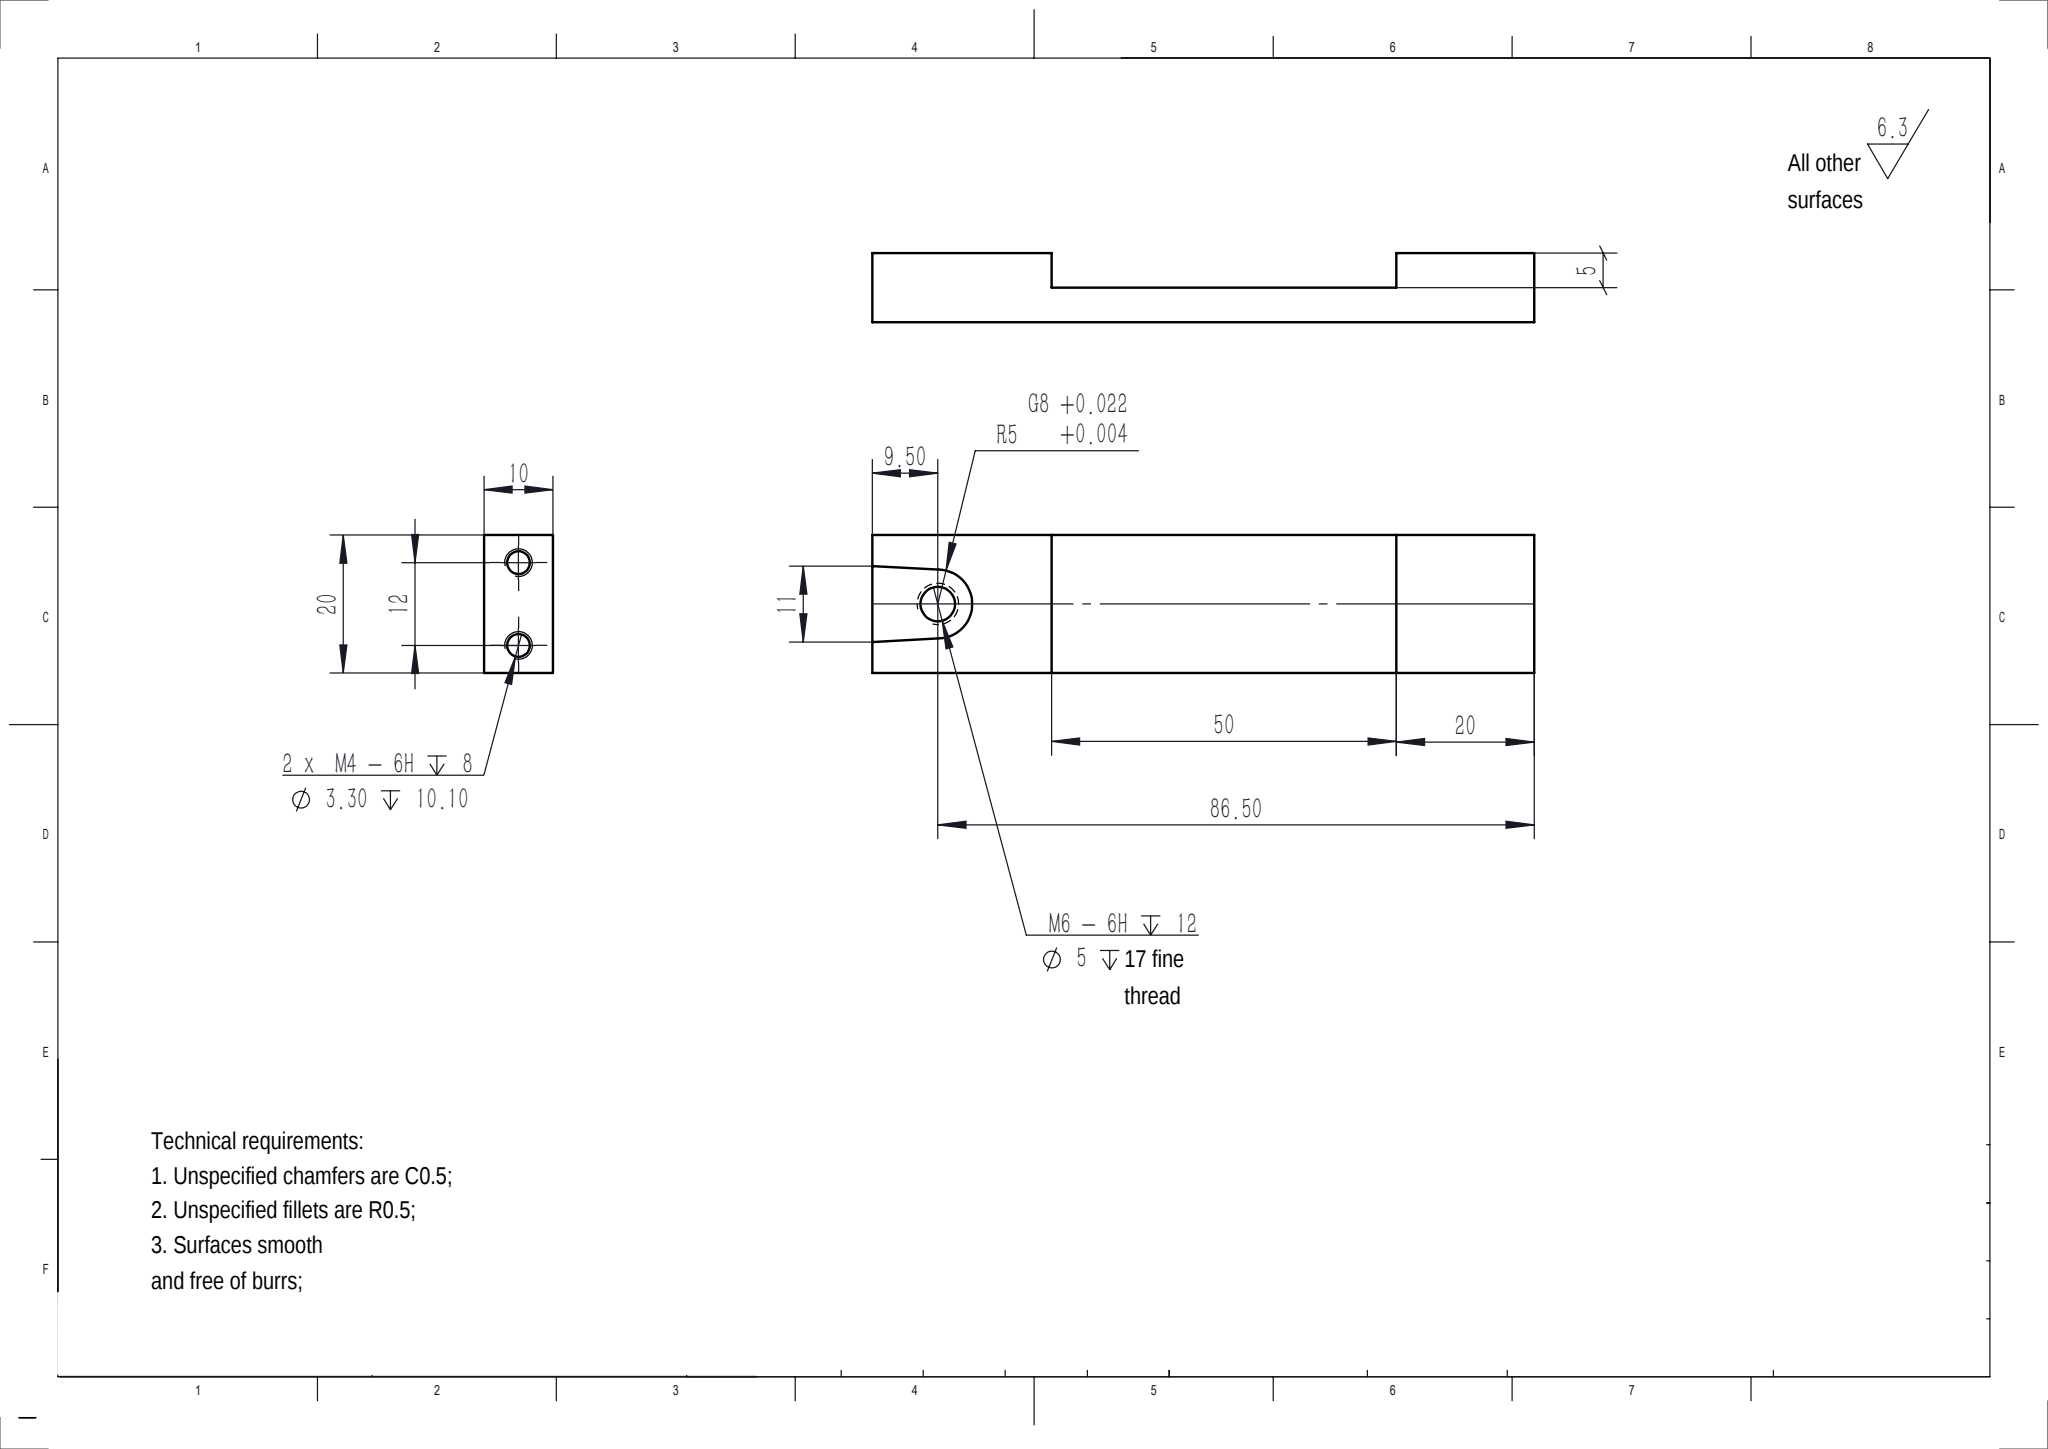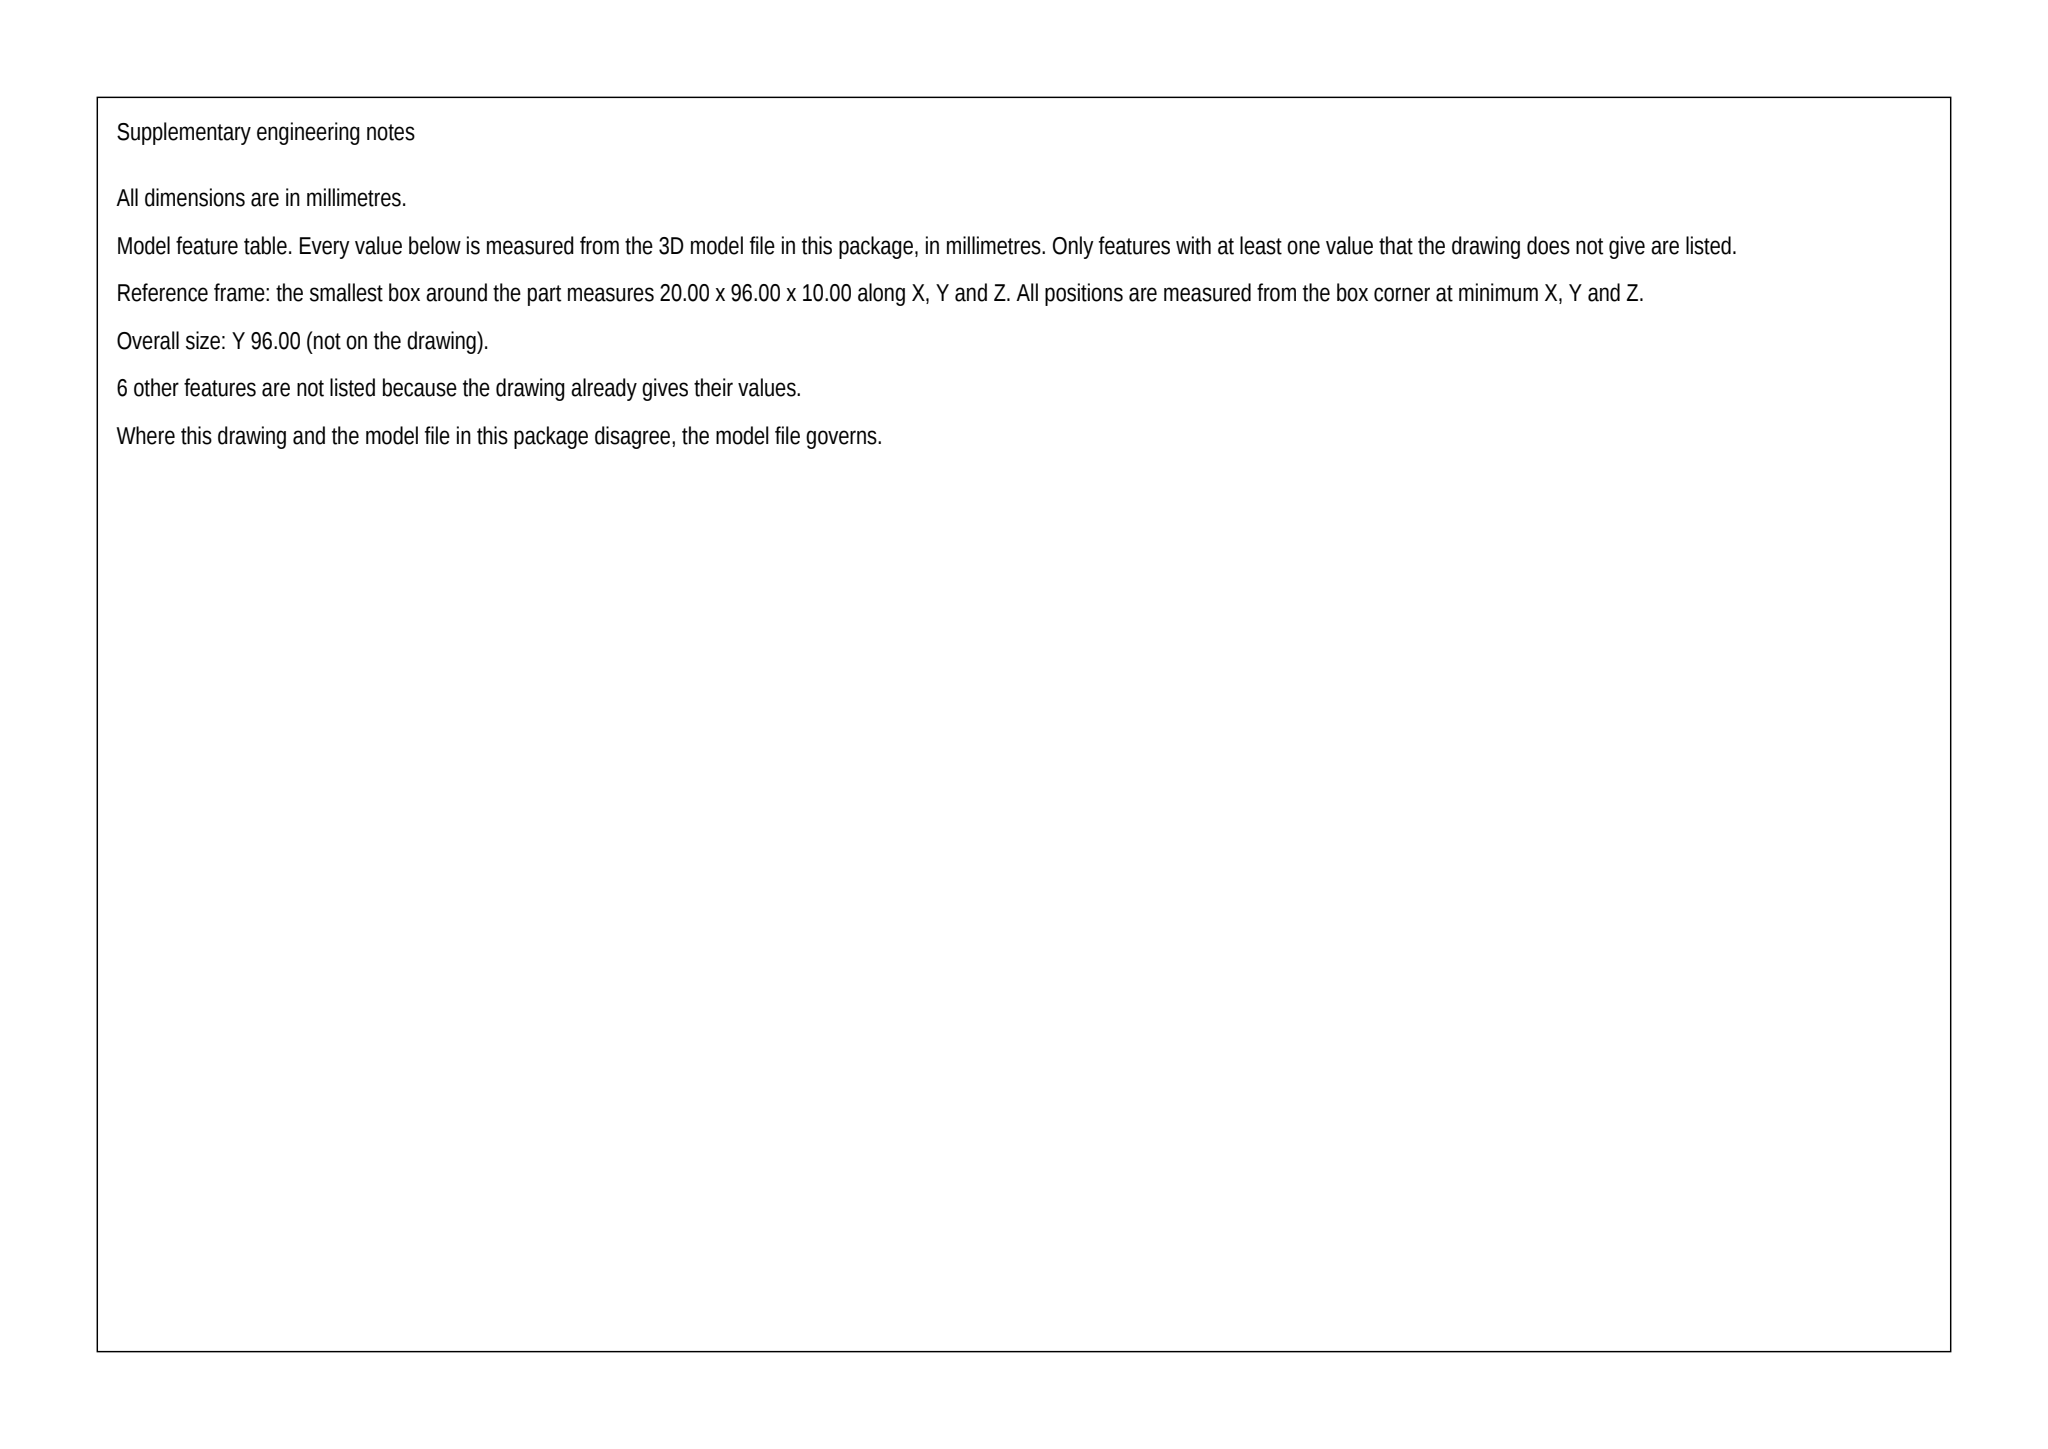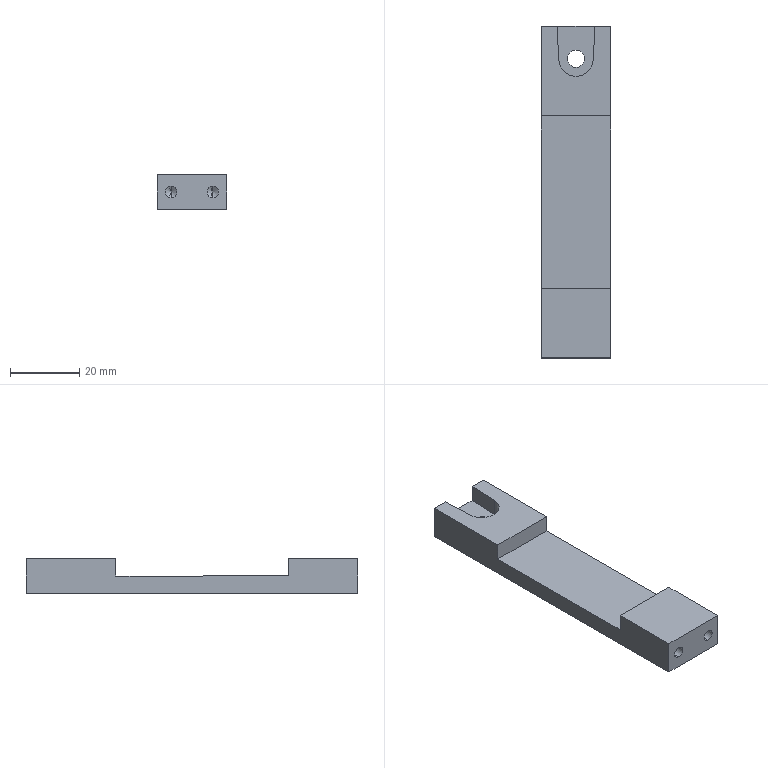Part | SolidWorks | mm | 1 solid | 24 faces | box 20 x 96 x 10 mm | volume 13228 mm3 | plane 13 | cylinder 7 | cone 4 | commonest cylinder face diameters 3.3 x4 5 x2 10 x1
build123d program:
from build123d import *

# Parameters (mm, degrees)
SKETCH1_W             = 20
SKETCH1_H             = 96
BOSS_EXTRUDE1_DEPTH   = 10
CUT_EXTRUDE1_DEPTH    = 5
M4_TAPPED_HOLE1_D     = 3.3
M4_TAPPED_HOLE1_DEPTH = 10.1
M4_TAPPED_HOLE1_TIP   = 0.9914
CUT_EXTRUDE3_DEPTH    = 5
M6_TAPPED_HOLE1_D     = 5
M6_TAPPED_HOLE1_DEPTH = 17
M6_TAPPED_HOLE1_TIP   = 1.502
SKETCH10_W            = 5
SKETCH10_H            = 50
CUT_EXTRUDE4_DEPTH    = 53.953


with BuildPart() as part:
    # Sketch1 → Boss-Extrude1 (new body)
    with BuildSketch(Plane.XY):
        Rectangle(SKETCH1_W, SKETCH1_H)
    extrude(amount=BOSS_EXTRUDE1_DEPTH)

    # Sketch2 → Cut-Extrude1 (cut)
    with BuildSketch(Plane.XY.offset(10)):
        with BuildLine():
            Line((-5, 48), (5, 48))
            Line((5, 48), (5, 38.5))
            ThreePointArc((5, 38.5), (0, 33.5), (-5, 38.5))
            Line((-5, 38.5), (-5, 48))
        make_face()
    extrude(amount=-CUT_EXTRUDE1_DEPTH, mode=Mode.SUBTRACT)

    # M4 Tapped Hole1
    with Locations(Plane(origin=(0, -48, 0), x_dir=(-1, 0, 0), z_dir=(0, -1, 0))):
        with Locations((6, -5), (-6, -5)):
            Hole(M4_TAPPED_HOLE1_D / 2, depth=M4_TAPPED_HOLE1_DEPTH)
            with Locations((0, 0, -(M4_TAPPED_HOLE1_DEPTH + M4_TAPPED_HOLE1_TIP / 2))):  # 118° drill point
                Cone(0, M4_TAPPED_HOLE1_D / 2, M4_TAPPED_HOLE1_TIP, mode=Mode.SUBTRACT)

    # Sketch7 → Cut-Extrude3 (cut)
    with BuildSketch(Plane.XY.offset(10)):
        Polygon((-5, 38.5), (-5.5, 48), (5.5, 48), (5, 38.5), align=None)
    extrude(amount=-CUT_EXTRUDE3_DEPTH, mode=Mode.SUBTRACT)

    # M6 Tapped Hole1
    with Locations(Plane(origin=(0, 0, 0), x_dir=(-1, 0, 0), z_dir=(0, 0, -1))):
        with Locations((0, 38.5)):
            Hole(M6_TAPPED_HOLE1_D / 2, depth=M6_TAPPED_HOLE1_DEPTH)
            with Locations((0, 0, -(M6_TAPPED_HOLE1_DEPTH + M6_TAPPED_HOLE1_TIP / 2))):  # 118° drill point
                Cone(0, M6_TAPPED_HOLE1_D / 2, M6_TAPPED_HOLE1_TIP, mode=Mode.SUBTRACT)

    # Sketch10 → Cut-Extrude4 (cut, through all)
    with BuildSketch(Plane.ZY.offset(10)):
        with Locations((7.5, -3)):
            Rectangle(SKETCH10_W, SKETCH10_H)
    extrude(amount=-CUT_EXTRUDE4_DEPTH, mode=Mode.SUBTRACT)


solid = part.part
STEP:
#1=CARTESIAN_POINT('',(-2.5,38.5,5.));
#2=VERTEX_POINT('',#1);
#3=CARTESIAN_POINT('',(2.5,38.5,5.));
#4=VERTEX_POINT('',#3);
#5=CARTESIAN_POINT('',(0.,38.5,5.));
#6=DIRECTION('',(0.,0.,1.));
#7=DIRECTION('',(1.,0.,0.));
#8=AXIS2_PLACEMENT_3D('',#5,#6,#7);
#9=CIRCLE('',#8,2.5);
#10=EDGE_CURVE('',#2,#4,#9,.T.);
#11=ORIENTED_EDGE('',*,*,#10,.T.);
#12=CARTESIAN_POINT('',(2.5,38.5,0.));
#13=VERTEX_POINT('',#12);
#14=CARTESIAN_POINT('',(2.5,38.5,0.));
#15=DIRECTION('',(0.,0.,-1.));
#16=VECTOR('',#15,1000.);
#17=LINE('',#14,#16);
#18=EDGE_CURVE('',#4,#13,#17,.T.);
#19=ORIENTED_EDGE('',*,*,#18,.T.);
#20=CARTESIAN_POINT('',(-2.5,38.5,0.));
#21=VERTEX_POINT('',#20);
#22=CARTESIAN_POINT('',(0.,38.5,0.));
#23=DIRECTION('',(0.,0.,-1.));
#24=DIRECTION('',(-1.,0.,0.));
#25=AXIS2_PLACEMENT_3D('',#22,#23,#24);
#26=CIRCLE('',#25,2.5);
#27=EDGE_CURVE('',#13,#21,#26,.T.);
#28=ORIENTED_EDGE('',*,*,#27,.T.);
#29=CARTESIAN_POINT('',(-2.5,38.5,0.));
#30=DIRECTION('',(0.,0.,-1.));
#31=VECTOR('',#30,1000.);
#32=LINE('',#29,#31);
#33=EDGE_CURVE('',#2,#21,#32,.T.);
#34=ORIENTED_EDGE('',*,*,#33,.F.);
#35=EDGE_LOOP('',(#11,#19,#28,#34));
#36=FACE_OUTER_BOUND('',#35,.T.);
#37=CARTESIAN_POINT('',(0.,38.5,0.));
#38=DIRECTION('',(0.,0.,-1.));
#39=DIRECTION('',(-1.,0.,0.));
#40=AXIS2_PLACEMENT_3D('',#37,#38,#39);
#41=CYLINDRICAL_SURFACE('',#40,2.5);
#42=ADVANCED_FACE('',(#36),#41,.F.);
#43=CARTESIAN_POINT('',(-6.,-37.9,6.65));
#44=VERTEX_POINT('',#43);
#45=CARTESIAN_POINT('',(-6.,-37.9,3.35));
#46=VERTEX_POINT('',#45);
#47=CARTESIAN_POINT('',(-6.,-37.9,5.));
#48=DIRECTION('',(0.,-1.,0.));
#49=DIRECTION('',(0.,0.,-1.));
#50=AXIS2_PLACEMENT_3D('',#47,#48,#49);
#51=CIRCLE('',#50,1.65);
#52=EDGE_CURVE('',#44,#46,#51,.T.);
#53=ORIENTED_EDGE('',*,*,#52,.F.);
#54=CARTESIAN_POINT('',(-6.,-48.,6.65));
#55=VERTEX_POINT('',#54);
#56=CARTESIAN_POINT('',(-6.,-48.,6.65));
#57=DIRECTION('',(0.,-1.,0.));
#58=VECTOR('',#57,1000.);
#59=LINE('',#56,#58);
#60=EDGE_CURVE('',#44,#55,#59,.T.);
#61=ORIENTED_EDGE('',*,*,#60,.T.);
#62=CARTESIAN_POINT('',(-6.,-48.,3.35));
#63=VERTEX_POINT('',#62);
#64=CARTESIAN_POINT('',(-6.,-48.,5.));
#65=DIRECTION('',(0.,-1.,0.));
#66=DIRECTION('',(0.,0.,-1.));
#67=AXIS2_PLACEMENT_3D('',#64,#65,#66);
#68=CIRCLE('',#67,1.65);
#69=EDGE_CURVE('',#55,#63,#68,.T.);
#70=ORIENTED_EDGE('',*,*,#69,.T.);
#71=CARTESIAN_POINT('',(-6.,-48.,3.35));
#72=DIRECTION('',(0.,-1.,0.));
#73=VECTOR('',#72,1000.);
#74=LINE('',#71,#73);
#75=EDGE_CURVE('',#46,#63,#74,.T.);
#76=ORIENTED_EDGE('',*,*,#75,.F.);
#77=EDGE_LOOP('',(#53,#61,#70,#76));
#78=FACE_OUTER_BOUND('',#77,.T.);
#79=CARTESIAN_POINT('',(-6.,-48.,5.));
#80=DIRECTION('',(0.,-1.,0.));
#81=DIRECTION('',(0.,0.,-1.));
#82=AXIS2_PLACEMENT_3D('',#79,#80,#81);
#83=CYLINDRICAL_SURFACE('',#82,1.65);
#84=ADVANCED_FACE('',(#78),#83,.F.);
#85=CARTESIAN_POINT('',(-6.,-36.909,5.));
#86=VERTEX_POINT('',#85);
#87=CARTESIAN_POINT('',(-6.,-37.9,3.35));
#88=DIRECTION('',(0.,-0.515,-0.8572));
#89=VECTOR('',#88,1000.);
#90=LINE('',#87,#89);
#91=EDGE_CURVE('',#86,#46,#90,.T.);
#92=ORIENTED_EDGE('',*,*,#91,.F.);
#93=CARTESIAN_POINT('',(-6.,-37.9,6.65));
#94=DIRECTION('',(0.,-0.515,0.8572));
#95=VECTOR('',#94,1000.);
#96=LINE('',#93,#95);
#97=EDGE_CURVE('',#86,#44,#96,.T.);
#98=ORIENTED_EDGE('',*,*,#97,.T.);
#99=ORIENTED_EDGE('',*,*,#52,.T.);
#100=EDGE_LOOP('',(#92,#98,#99));
#101=FACE_OUTER_BOUND('',#100,.T.);
#102=CARTESIAN_POINT('',(-6.,-37.9,5.));
#103=DIRECTION('',(0.,-1.,0.));
#104=DIRECTION('',(0.,0.,-1.));
#105=AXIS2_PLACEMENT_3D('',#102,#103,#104);
#106=CONICAL_SURFACE('',#105,1.65,1.03);
#107=ADVANCED_FACE('',(#101),#106,.F.);
#108=CARTESIAN_POINT('',(6.,-37.9,6.65));
#109=VERTEX_POINT('',#108);
#110=CARTESIAN_POINT('',(6.,-37.9,3.35));
#111=VERTEX_POINT('',#110);
#112=CARTESIAN_POINT('',(6.,-37.9,5.));
#113=DIRECTION('',(0.,-1.,0.));
#114=DIRECTION('',(0.,0.,-1.));
#115=AXIS2_PLACEMENT_3D('',#112,#113,#114);
#116=CIRCLE('',#115,1.65);
#117=EDGE_CURVE('',#109,#111,#116,.T.);
#118=ORIENTED_EDGE('',*,*,#117,.F.);
#119=CARTESIAN_POINT('',(6.,-48.,6.65));
#120=VERTEX_POINT('',#119);
#121=CARTESIAN_POINT('',(6.,-48.,6.65));
#122=DIRECTION('',(0.,-1.,0.));
#123=VECTOR('',#122,1000.);
#124=LINE('',#121,#123);
#125=EDGE_CURVE('',#109,#120,#124,.T.);
#126=ORIENTED_EDGE('',*,*,#125,.T.);
#127=CARTESIAN_POINT('',(6.,-48.,3.35));
#128=VERTEX_POINT('',#127);
#129=CARTESIAN_POINT('',(6.,-48.,5.));
#130=DIRECTION('',(0.,-1.,0.));
#131=DIRECTION('',(0.,0.,-1.));
#132=AXIS2_PLACEMENT_3D('',#129,#130,#131);
#133=CIRCLE('',#132,1.65);
#134=EDGE_CURVE('',#120,#128,#133,.T.);
#135=ORIENTED_EDGE('',*,*,#134,.T.);
#136=CARTESIAN_POINT('',(6.,-48.,3.35));
#137=DIRECTION('',(0.,-1.,0.));
#138=VECTOR('',#137,1000.);
#139=LINE('',#136,#138);
#140=EDGE_CURVE('',#111,#128,#139,.T.);
#141=ORIENTED_EDGE('',*,*,#140,.F.);
#142=EDGE_LOOP('',(#118,#126,#135,#141));
#143=FACE_OUTER_BOUND('',#142,.T.);
#144=CARTESIAN_POINT('',(6.,-48.,5.));
#145=DIRECTION('',(0.,-1.,0.));
#146=DIRECTION('',(0.,0.,-1.));
#147=AXIS2_PLACEMENT_3D('',#144,#145,#146);
#148=CYLINDRICAL_SURFACE('',#147,1.65);
#149=ADVANCED_FACE('',(#143),#148,.F.);
#150=CARTESIAN_POINT('',(6.,-36.909,5.));
#151=VERTEX_POINT('',#150);
#152=CARTESIAN_POINT('',(6.,-37.9,3.35));
#153=DIRECTION('',(0.,-0.515,-0.8572));
#154=VECTOR('',#153,1000.);
#155=LINE('',#152,#154);
#156=EDGE_CURVE('',#151,#111,#155,.T.);
#157=ORIENTED_EDGE('',*,*,#156,.F.);
#158=CARTESIAN_POINT('',(6.,-37.9,6.65));
#159=DIRECTION('',(0.,-0.515,0.8572));
#160=VECTOR('',#159,1000.);
#161=LINE('',#158,#160);
#162=EDGE_CURVE('',#151,#109,#161,.T.);
#163=ORIENTED_EDGE('',*,*,#162,.T.);
#164=ORIENTED_EDGE('',*,*,#117,.T.);
#165=EDGE_LOOP('',(#157,#163,#164));
#166=FACE_OUTER_BOUND('',#165,.T.);
#167=CARTESIAN_POINT('',(6.,-37.9,5.));
#168=DIRECTION('',(0.,-1.,0.));
#169=DIRECTION('',(0.,0.,-1.));
#170=AXIS2_PLACEMENT_3D('',#167,#168,#169);
#171=CONICAL_SURFACE('',#170,1.65,1.03);
#172=ADVANCED_FACE('',(#166),#171,.F.);
#173=CARTESIAN_POINT('',(10.,-28.,10.));
#174=VERTEX_POINT('',#173);
#175=CARTESIAN_POINT('',(-10.,-28.,10.));
#176=VERTEX_POINT('',#175);
#177=CARTESIAN_POINT('',(10.,-28.,10.));
#178=DIRECTION('',(-1.,-0.,0.));
#179=VECTOR('',#178,1000.);
#180=LINE('',#177,#179);
#181=EDGE_CURVE('',#174,#176,#180,.T.);
#182=ORIENTED_EDGE('',*,*,#181,.T.);
#183=CARTESIAN_POINT('',(-10.,-48.,10.));
#184=VERTEX_POINT('',#183);
#185=CARTESIAN_POINT('',(-10.,48.,10.));
#186=DIRECTION('',(0.,-1.,0.));
#187=VECTOR('',#186,1000.);
#188=LINE('',#185,#187);
#189=EDGE_CURVE('',#176,#184,#188,.T.);
#190=ORIENTED_EDGE('',*,*,#189,.T.);
#191=CARTESIAN_POINT('',(10.,-48.,10.));
#192=VERTEX_POINT('',#191);
#193=CARTESIAN_POINT('',(-10.,-48.,10.));
#194=DIRECTION('',(1.,0.,0.));
#195=VECTOR('',#194,1000.);
#196=LINE('',#193,#195);
#197=EDGE_CURVE('',#184,#192,#196,.T.);
#198=ORIENTED_EDGE('',*,*,#197,.T.);
#199=CARTESIAN_POINT('',(10.,48.,10.));
#200=DIRECTION('',(-0.,1.,0.));
#201=VECTOR('',#200,1000.);
#202=LINE('',#199,#201);
#203=EDGE_CURVE('',#192,#174,#202,.T.);
#204=ORIENTED_EDGE('',*,*,#203,.T.);
#205=EDGE_LOOP('',(#182,#190,#198,#204));
#206=FACE_OUTER_BOUND('',#205,.T.);
#207=CARTESIAN_POINT('',(0.,0.,10.));
#208=DIRECTION('',(0.,0.,1.));
#209=DIRECTION('',(1.,0.,0.));
#210=AXIS2_PLACEMENT_3D('',#207,#208,#209);
#211=PLANE('',#210);
#212=ADVANCED_FACE('',(#206),#211,.T.);
#213=CARTESIAN_POINT('',(10.,22.,5.));
#214=VERTEX_POINT('',#213);
#215=CARTESIAN_POINT('',(10.,-28.,5.));
#216=VERTEX_POINT('',#215);
#217=CARTESIAN_POINT('',(10.,22.,5.));
#218=DIRECTION('',(0.,-1.,0.));
#219=VECTOR('',#218,1000.);
#220=LINE('',#217,#219);
#221=EDGE_CURVE('',#214,#216,#220,.T.);
#222=ORIENTED_EDGE('',*,*,#221,.T.);
#223=CARTESIAN_POINT('',(10.,-28.,10.));
#224=DIRECTION('',(0.,0.,1.));
#225=VECTOR('',#224,1000.);
#226=LINE('',#223,#225);
#227=EDGE_CURVE('',#216,#174,#226,.T.);
#228=ORIENTED_EDGE('',*,*,#227,.T.);
#229=ORIENTED_EDGE('',*,*,#203,.F.);
#230=CARTESIAN_POINT('',(10.,-48.,0.));
#231=VERTEX_POINT('',#230);
#232=CARTESIAN_POINT('',(10.,-48.,10.));
#233=DIRECTION('',(0.,0.,-1.));
#234=VECTOR('',#233,1000.);
#235=LINE('',#232,#234);
#236=EDGE_CURVE('',#192,#231,#235,.T.);
#237=ORIENTED_EDGE('',*,*,#236,.T.);
#238=CARTESIAN_POINT('',(10.,48.,0.));
#239=VERTEX_POINT('',#238);
#240=CARTESIAN_POINT('',(10.,48.,0.));
#241=DIRECTION('',(-0.,1.,0.));
#242=VECTOR('',#241,1000.);
#243=LINE('',#240,#242);
#244=EDGE_CURVE('',#231,#239,#243,.T.);
#245=ORIENTED_EDGE('',*,*,#244,.T.);
#246=CARTESIAN_POINT('',(10.,48.,10.));
#247=VERTEX_POINT('',#246);
#248=CARTESIAN_POINT('',(10.,48.,10.));
#249=DIRECTION('',(0.,0.,-1.));
#250=VECTOR('',#249,1000.);
#251=LINE('',#248,#250);
#252=EDGE_CURVE('',#247,#239,#251,.T.);
#253=ORIENTED_EDGE('',*,*,#252,.F.);
#254=CARTESIAN_POINT('',(10.,22.,10.));
#255=VERTEX_POINT('',#254);
#256=CARTESIAN_POINT('',(10.,48.,10.));
#257=DIRECTION('',(-0.,1.,0.));
#258=VECTOR('',#257,1000.);
#259=LINE('',#256,#258);
#260=EDGE_CURVE('',#255,#247,#259,.T.);
#261=ORIENTED_EDGE('',*,*,#260,.F.);
#262=CARTESIAN_POINT('',(10.,22.,10.));
#263=DIRECTION('',(0.,0.,-1.));
#264=VECTOR('',#263,1000.);
#265=LINE('',#262,#264);
#266=EDGE_CURVE('',#255,#214,#265,.T.);
#267=ORIENTED_EDGE('',*,*,#266,.T.);
#268=EDGE_LOOP('',(#222,#228,#229,#237,#245,#253,#261,#267));
#269=FACE_OUTER_BOUND('',#268,.T.);
#270=CARTESIAN_POINT('',(10.,48.,10.));
#271=DIRECTION('',(-1.,-0.,0.));
#272=DIRECTION('',(0.,-1.,0.));
#273=AXIS2_PLACEMENT_3D('',#270,#271,#272);
#274=PLANE('',#273);
#275=ADVANCED_FACE('',(#269),#274,.F.);
#276=CARTESIAN_POINT('',(5.5,48.,5.));
#277=VERTEX_POINT('',#276);
#278=CARTESIAN_POINT('',(-5.5,48.,5.));
#279=VERTEX_POINT('',#278);
#280=CARTESIAN_POINT('',(-5.,48.,5.));
#281=DIRECTION('',(-1.,0.,0.));
#282=VECTOR('',#281,1000.);
#283=LINE('',#280,#282);
#284=EDGE_CURVE('',#277,#279,#283,.T.);
#285=ORIENTED_EDGE('',*,*,#284,.F.);
#286=CARTESIAN_POINT('',(5.5,48.,10.));
#287=VERTEX_POINT('',#286);
#288=CARTESIAN_POINT('',(5.5,48.,-9.534));
#289=DIRECTION('',(0.,0.,1.));
#290=VECTOR('',#289,1000.);
#291=LINE('',#288,#290);
#292=EDGE_CURVE('',#277,#287,#291,.T.);
#293=ORIENTED_EDGE('',*,*,#292,.T.);
#294=CARTESIAN_POINT('',(-10.,48.,10.));
#295=DIRECTION('',(-1.,0.,0.));
#296=VECTOR('',#295,1000.);
#297=LINE('',#294,#296);
#298=EDGE_CURVE('',#247,#287,#297,.T.);
#299=ORIENTED_EDGE('',*,*,#298,.F.);
#300=ORIENTED_EDGE('',*,*,#252,.T.);
#301=CARTESIAN_POINT('',(-10.,48.,0.));
#302=VERTEX_POINT('',#301);
#303=CARTESIAN_POINT('',(-10.,48.,0.));
#304=DIRECTION('',(-1.,0.,0.));
#305=VECTOR('',#304,1000.);
#306=LINE('',#303,#305);
#307=EDGE_CURVE('',#239,#302,#306,.T.);
#308=ORIENTED_EDGE('',*,*,#307,.T.);
#309=CARTESIAN_POINT('',(-10.,48.,10.));
#310=VERTEX_POINT('',#309);
#311=CARTESIAN_POINT('',(-10.,48.,10.));
#312=DIRECTION('',(0.,0.,-1.));
#313=VECTOR('',#312,1000.);
#314=LINE('',#311,#313);
#315=EDGE_CURVE('',#310,#302,#314,.T.);
#316=ORIENTED_EDGE('',*,*,#315,.F.);
#317=CARTESIAN_POINT('',(-5.5,48.,10.));
#318=VERTEX_POINT('',#317);
#319=CARTESIAN_POINT('',(-10.,48.,10.));
#320=DIRECTION('',(-1.,0.,0.));
#321=VECTOR('',#320,1000.);
#322=LINE('',#319,#321);
#323=EDGE_CURVE('',#318,#310,#322,.T.);
#324=ORIENTED_EDGE('',*,*,#323,.F.);
#325=CARTESIAN_POINT('',(-5.5,48.,-9.534));
#326=DIRECTION('',(0.,0.,1.));
#327=VECTOR('',#326,1000.);
#328=LINE('',#325,#327);
#329=EDGE_CURVE('',#279,#318,#328,.T.);
#330=ORIENTED_EDGE('',*,*,#329,.F.);
#331=EDGE_LOOP('',(#285,#293,#299,#300,#308,#316,#324,#330));
#332=FACE_OUTER_BOUND('',#331,.T.);
#333=CARTESIAN_POINT('',(-10.,48.,10.));
#334=DIRECTION('',(0.,-1.,0.));
#335=DIRECTION('',(0.,0.,-1.));
#336=AXIS2_PLACEMENT_3D('',#333,#334,#335);
#337=PLANE('',#336);
#338=ADVANCED_FACE('',(#332),#337,.F.);
#339=ORIENTED_EDGE('',*,*,#189,.F.);
#340=CARTESIAN_POINT('',(-10.,-28.,5.));
#341=VERTEX_POINT('',#340);
#342=CARTESIAN_POINT('',(-10.,-28.,10.));
#343=DIRECTION('',(0.,0.,1.));
#344=VECTOR('',#343,1000.);
#345=LINE('',#342,#344);
#346=EDGE_CURVE('',#341,#176,#345,.T.);
#347=ORIENTED_EDGE('',*,*,#346,.F.);
#348=CARTESIAN_POINT('',(-10.,22.,5.));
#349=VERTEX_POINT('',#348);
#350=CARTESIAN_POINT('',(-10.,22.,5.));
#351=DIRECTION('',(0.,-1.,0.));
#352=VECTOR('',#351,1000.);
#353=LINE('',#350,#352);
#354=EDGE_CURVE('',#349,#341,#353,.T.);
#355=ORIENTED_EDGE('',*,*,#354,.F.);
#356=CARTESIAN_POINT('',(-10.,22.,10.));
#357=VERTEX_POINT('',#356);
#358=CARTESIAN_POINT('',(-10.,22.,10.));
#359=DIRECTION('',(0.,0.,-1.));
#360=VECTOR('',#359,1000.);
#361=LINE('',#358,#360);
#362=EDGE_CURVE('',#357,#349,#361,.T.);
#363=ORIENTED_EDGE('',*,*,#362,.F.);
#364=CARTESIAN_POINT('',(-10.,48.,10.));
#365=DIRECTION('',(0.,-1.,0.));
#366=VECTOR('',#365,1000.);
#367=LINE('',#364,#366);
#368=EDGE_CURVE('',#310,#357,#367,.T.);
#369=ORIENTED_EDGE('',*,*,#368,.F.);
#370=ORIENTED_EDGE('',*,*,#315,.T.);
#371=CARTESIAN_POINT('',(-10.,-48.,0.));
#372=VERTEX_POINT('',#371);
#373=CARTESIAN_POINT('',(-10.,48.,0.));
#374=DIRECTION('',(0.,-1.,0.));
#375=VECTOR('',#374,1000.);
#376=LINE('',#373,#375);
#377=EDGE_CURVE('',#302,#372,#376,.T.);
#378=ORIENTED_EDGE('',*,*,#377,.T.);
#379=CARTESIAN_POINT('',(-10.,-48.,10.));
#380=DIRECTION('',(0.,0.,-1.));
#381=VECTOR('',#380,1000.);
#382=LINE('',#379,#381);
#383=EDGE_CURVE('',#184,#372,#382,.T.);
#384=ORIENTED_EDGE('',*,*,#383,.F.);
#385=EDGE_LOOP('',(#339,#347,#355,#363,#369,#370,#378,#384));
#386=FACE_OUTER_BOUND('',#385,.T.);
#387=CARTESIAN_POINT('',(-10.,48.,10.));
#388=DIRECTION('',(1.,0.,0.));
#389=DIRECTION('',(-0.,1.,0.));
#390=AXIS2_PLACEMENT_3D('',#387,#388,#389);
#391=PLANE('',#390);
#392=ADVANCED_FACE('',(#386),#391,.F.);
#393=CARTESIAN_POINT('',(-6.,-48.,5.));
#394=DIRECTION('',(0.,-1.,0.));
#395=DIRECTION('',(0.,0.,-1.));
#396=AXIS2_PLACEMENT_3D('',#393,#394,#395);
#397=CIRCLE('',#396,1.65);
#398=EDGE_CURVE('',#63,#55,#397,.T.);
#399=ORIENTED_EDGE('',*,*,#398,.F.);
#400=ORIENTED_EDGE('',*,*,#69,.F.);
#401=EDGE_LOOP('',(#399,#400));
#402=FACE_BOUND('',#401,.T.);
#403=CARTESIAN_POINT('',(6.,-48.,5.));
#404=DIRECTION('',(0.,-1.,0.));
#405=DIRECTION('',(0.,0.,-1.));
#406=AXIS2_PLACEMENT_3D('',#403,#404,#405);
#407=CIRCLE('',#406,1.65);
#408=EDGE_CURVE('',#128,#120,#407,.T.);
#409=ORIENTED_EDGE('',*,*,#408,.F.);
#410=ORIENTED_EDGE('',*,*,#134,.F.);
#411=EDGE_LOOP('',(#409,#410));
#412=FACE_BOUND('',#411,.T.);
#413=CARTESIAN_POINT('',(-10.,-48.,0.));
#414=DIRECTION('',(1.,0.,0.));
#415=VECTOR('',#414,1000.);
#416=LINE('',#413,#415);
#417=EDGE_CURVE('',#372,#231,#416,.T.);
#418=ORIENTED_EDGE('',*,*,#417,.T.);
#419=ORIENTED_EDGE('',*,*,#236,.F.);
#420=ORIENTED_EDGE('',*,*,#197,.F.);
#421=ORIENTED_EDGE('',*,*,#383,.T.);
#422=EDGE_LOOP('',(#418,#419,#420,#421));
#423=FACE_OUTER_BOUND('',#422,.T.);
#424=CARTESIAN_POINT('',(-10.,-48.,10.));
#425=DIRECTION('',(0.,1.,0.));
#426=DIRECTION('',(0.,0.,1.));
#427=AXIS2_PLACEMENT_3D('',#424,#425,#426);
#428=PLANE('',#427);
#429=ADVANCED_FACE('',(#402,#412,#423),#428,.F.);
#430=CARTESIAN_POINT('',(10.,22.,10.));
#431=DIRECTION('',(-1.,-0.,0.));
#432=VECTOR('',#431,1000.);
#433=LINE('',#430,#432);
#434=EDGE_CURVE('',#255,#357,#433,.T.);
#435=ORIENTED_EDGE('',*,*,#434,.F.);
#436=ORIENTED_EDGE('',*,*,#260,.T.);
#437=ORIENTED_EDGE('',*,*,#298,.T.);
#438=CARTESIAN_POINT('',(5.,38.5,10.));
#439=VERTEX_POINT('',#438);
#440=CARTESIAN_POINT('',(5.5,48.,10.));
#441=DIRECTION('',(0.05256,0.9986,0.));
#442=VECTOR('',#441,1000.);
#443=LINE('',#440,#442);
#444=EDGE_CURVE('',#439,#287,#443,.T.);
#445=ORIENTED_EDGE('',*,*,#444,.F.);
#446=CARTESIAN_POINT('',(-5.,38.5,10.));
#447=VERTEX_POINT('',#446);
#448=CARTESIAN_POINT('',(-0.,38.5,10.));
#449=DIRECTION('',(0.,0.,1.));
#450=DIRECTION('',(1.,0.,0.));
#451=AXIS2_PLACEMENT_3D('',#448,#449,#450);
#452=CIRCLE('',#451,5.);
#453=EDGE_CURVE('',#447,#439,#452,.T.);
#454=ORIENTED_EDGE('',*,*,#453,.F.);
#455=CARTESIAN_POINT('',(-5.,38.5,10.));
#456=DIRECTION('',(0.05256,-0.9986,0.));
#457=VECTOR('',#456,1000.);
#458=LINE('',#455,#457);
#459=EDGE_CURVE('',#318,#447,#458,.T.);
#460=ORIENTED_EDGE('',*,*,#459,.F.);
#461=ORIENTED_EDGE('',*,*,#323,.T.);
#462=ORIENTED_EDGE('',*,*,#368,.T.);
#463=EDGE_LOOP('',(#435,#436,#437,#445,#454,#460,#461,#462));
#464=FACE_OUTER_BOUND('',#463,.T.);
#465=CARTESIAN_POINT('',(0.,0.,10.));
#466=DIRECTION('',(0.,0.,1.));
#467=DIRECTION('',(1.,0.,0.));
#468=AXIS2_PLACEMENT_3D('',#465,#466,#467);
#469=PLANE('',#468);
#470=ADVANCED_FACE('',(#464),#469,.T.);
#471=CARTESIAN_POINT('',(0.,38.5,0.));
#472=DIRECTION('',(0.,0.,-1.));
#473=DIRECTION('',(-1.,0.,0.));
#474=AXIS2_PLACEMENT_3D('',#471,#472,#473);
#475=CIRCLE('',#474,2.5);
#476=EDGE_CURVE('',#21,#13,#475,.T.);
#477=ORIENTED_EDGE('',*,*,#476,.F.);
#478=ORIENTED_EDGE('',*,*,#27,.F.);
#479=EDGE_LOOP('',(#477,#478));
#480=FACE_BOUND('',#479,.T.);
#481=ORIENTED_EDGE('',*,*,#244,.F.);
#482=ORIENTED_EDGE('',*,*,#417,.F.);
#483=ORIENTED_EDGE('',*,*,#377,.F.);
#484=ORIENTED_EDGE('',*,*,#307,.F.);
#485=EDGE_LOOP('',(#481,#482,#483,#484));
#486=FACE_OUTER_BOUND('',#485,.T.);
#487=CARTESIAN_POINT('',(0.,0.,0.));
#488=DIRECTION('',(0.,0.,1.));
#489=DIRECTION('',(1.,0.,0.));
#490=AXIS2_PLACEMENT_3D('',#487,#488,#489);
#491=PLANE('',#490);
#492=ADVANCED_FACE('',(#480,#486),#491,.F.);
#493=ORIENTED_EDGE('',*,*,#453,.T.);
#494=CARTESIAN_POINT('',(5.,38.5,5.));
#495=VERTEX_POINT('',#494);
#496=CARTESIAN_POINT('',(5.,38.5,5.));
#497=DIRECTION('',(0.,0.,1.));
#498=VECTOR('',#497,1000.);
#499=LINE('',#496,#498);
#500=EDGE_CURVE('',#495,#439,#499,.T.);
#501=ORIENTED_EDGE('',*,*,#500,.F.);
#502=CARTESIAN_POINT('',(-5.,38.5,5.));
#503=VERTEX_POINT('',#502);
#504=CARTESIAN_POINT('',(-0.,38.5,5.));
#505=DIRECTION('',(0.,0.,1.));
#506=DIRECTION('',(1.,0.,0.));
#507=AXIS2_PLACEMENT_3D('',#504,#505,#506);
#508=CIRCLE('',#507,5.);
#509=EDGE_CURVE('',#503,#495,#508,.T.);
#510=ORIENTED_EDGE('',*,*,#509,.F.);
#511=CARTESIAN_POINT('',(-5.,38.5,5.));
#512=DIRECTION('',(0.,0.,1.));
#513=VECTOR('',#512,1000.);
#514=LINE('',#511,#513);
#515=EDGE_CURVE('',#503,#447,#514,.T.);
#516=ORIENTED_EDGE('',*,*,#515,.T.);
#517=EDGE_LOOP('',(#493,#501,#510,#516));
#518=FACE_OUTER_BOUND('',#517,.T.);
#519=CARTESIAN_POINT('',(-0.,38.5,5.));
#520=DIRECTION('',(0.,0.,1.));
#521=DIRECTION('',(1.,0.,0.));
#522=AXIS2_PLACEMENT_3D('',#519,#520,#521);
#523=CYLINDRICAL_SURFACE('',#522,5.);
#524=ADVANCED_FACE('',(#518),#523,.F.);
#525=ORIENTED_EDGE('',*,*,#10,.F.);
#526=CARTESIAN_POINT('',(0.,38.5,5.));
#527=DIRECTION('',(0.,0.,1.));
#528=DIRECTION('',(1.,0.,0.));
#529=AXIS2_PLACEMENT_3D('',#526,#527,#528);
#530=CIRCLE('',#529,2.5);
#531=EDGE_CURVE('',#4,#2,#530,.T.);
#532=ORIENTED_EDGE('',*,*,#531,.F.);
#533=EDGE_LOOP('',(#525,#532));
#534=FACE_BOUND('',#533,.T.);
#535=ORIENTED_EDGE('',*,*,#509,.T.);
#536=CARTESIAN_POINT('',(5.5,48.,5.));
#537=DIRECTION('',(-0.05256,-0.9986,0.));
#538=VECTOR('',#537,1000.);
#539=LINE('',#536,#538);
#540=EDGE_CURVE('',#277,#495,#539,.T.);
#541=ORIENTED_EDGE('',*,*,#540,.F.);
#542=ORIENTED_EDGE('',*,*,#284,.T.);
#543=CARTESIAN_POINT('',(-5.,38.5,5.));
#544=DIRECTION('',(-0.05256,0.9986,0.));
#545=VECTOR('',#544,1000.);
#546=LINE('',#543,#545);
#547=EDGE_CURVE('',#503,#279,#546,.T.);
#548=ORIENTED_EDGE('',*,*,#547,.F.);
#549=EDGE_LOOP('',(#535,#541,#542,#548));
#550=FACE_OUTER_BOUND('',#549,.T.);
#551=CARTESIAN_POINT('',(-0.,38.5,5.));
#552=DIRECTION('',(0.,0.,1.));
#553=DIRECTION('',(1.,0.,0.));
#554=AXIS2_PLACEMENT_3D('',#551,#552,#553);
#555=PLANE('',#554);
#556=ADVANCED_FACE('',(#534,#550),#555,.T.);
#557=ORIENTED_EDGE('',*,*,#162,.F.);
#558=ORIENTED_EDGE('',*,*,#156,.T.);
#559=CARTESIAN_POINT('',(6.,-37.9,5.));
#560=DIRECTION('',(0.,-1.,0.));
#561=DIRECTION('',(0.,0.,-1.));
#562=AXIS2_PLACEMENT_3D('',#559,#560,#561);
#563=CIRCLE('',#562,1.65);
#564=EDGE_CURVE('',#111,#109,#563,.T.);
#565=ORIENTED_EDGE('',*,*,#564,.T.);
#566=EDGE_LOOP('',(#557,#558,#565));
#567=FACE_OUTER_BOUND('',#566,.T.);
#568=CARTESIAN_POINT('',(6.,-37.9,5.));
#569=DIRECTION('',(0.,-1.,0.));
#570=DIRECTION('',(0.,0.,-1.));
#571=AXIS2_PLACEMENT_3D('',#568,#569,#570);
#572=CONICAL_SURFACE('',#571,1.65,1.03);
#573=ADVANCED_FACE('',(#567),#572,.F.);
#574=ORIENTED_EDGE('',*,*,#125,.F.);
#575=ORIENTED_EDGE('',*,*,#564,.F.);
#576=ORIENTED_EDGE('',*,*,#140,.T.);
#577=ORIENTED_EDGE('',*,*,#408,.T.);
#578=EDGE_LOOP('',(#574,#575,#576,#577));
#579=FACE_OUTER_BOUND('',#578,.T.);
#580=CARTESIAN_POINT('',(6.,-48.,5.));
#581=DIRECTION('',(0.,-1.,0.));
#582=DIRECTION('',(0.,0.,-1.));
#583=AXIS2_PLACEMENT_3D('',#580,#581,#582);
#584=CYLINDRICAL_SURFACE('',#583,1.65);
#585=ADVANCED_FACE('',(#579),#584,.F.);
#586=ORIENTED_EDGE('',*,*,#97,.F.);
#587=ORIENTED_EDGE('',*,*,#91,.T.);
#588=CARTESIAN_POINT('',(-6.,-37.9,5.));
#589=DIRECTION('',(0.,-1.,0.));
#590=DIRECTION('',(0.,0.,-1.));
#591=AXIS2_PLACEMENT_3D('',#588,#589,#590);
#592=CIRCLE('',#591,1.65);
#593=EDGE_CURVE('',#46,#44,#592,.T.);
#594=ORIENTED_EDGE('',*,*,#593,.T.);
#595=EDGE_LOOP('',(#586,#587,#594));
#596=FACE_OUTER_BOUND('',#595,.T.);
#597=CARTESIAN_POINT('',(-6.,-37.9,5.));
#598=DIRECTION('',(0.,-1.,0.));
#599=DIRECTION('',(0.,0.,-1.));
#600=AXIS2_PLACEMENT_3D('',#597,#598,#599);
#601=CONICAL_SURFACE('',#600,1.65,1.03);
#602=ADVANCED_FACE('',(#596),#601,.F.);
#603=ORIENTED_EDGE('',*,*,#60,.F.);
#604=ORIENTED_EDGE('',*,*,#593,.F.);
#605=ORIENTED_EDGE('',*,*,#75,.T.);
#606=ORIENTED_EDGE('',*,*,#398,.T.);
#607=EDGE_LOOP('',(#603,#604,#605,#606));
#608=FACE_OUTER_BOUND('',#607,.T.);
#609=CARTESIAN_POINT('',(-6.,-48.,5.));
#610=DIRECTION('',(0.,-1.,0.));
#611=DIRECTION('',(0.,0.,-1.));
#612=AXIS2_PLACEMENT_3D('',#609,#610,#611);
#613=CYLINDRICAL_SURFACE('',#612,1.65);
#614=ADVANCED_FACE('',(#608),#613,.F.);
#615=ORIENTED_EDGE('',*,*,#540,.T.);
#616=ORIENTED_EDGE('',*,*,#500,.T.);
#617=ORIENTED_EDGE('',*,*,#444,.T.);
#618=ORIENTED_EDGE('',*,*,#292,.F.);
#619=EDGE_LOOP('',(#615,#616,#617,#618));
#620=FACE_OUTER_BOUND('',#619,.T.);
#621=CARTESIAN_POINT('',(5.5,48.,-9.534));
#622=DIRECTION('',(0.9986,-0.05256,0.));
#623=DIRECTION('',(0.05256,0.9986,0.));
#624=AXIS2_PLACEMENT_3D('',#621,#622,#623);
#625=PLANE('',#624);
#626=ADVANCED_FACE('',(#620),#625,.F.);
#627=ORIENTED_EDGE('',*,*,#547,.T.);
#628=ORIENTED_EDGE('',*,*,#329,.T.);
#629=ORIENTED_EDGE('',*,*,#459,.T.);
#630=ORIENTED_EDGE('',*,*,#515,.F.);
#631=EDGE_LOOP('',(#627,#628,#629,#630));
#632=FACE_OUTER_BOUND('',#631,.T.);
#633=CARTESIAN_POINT('',(-5.,38.5,-9.534));
#634=DIRECTION('',(-0.9986,-0.05256,0.));
#635=DIRECTION('',(0.05256,-0.9986,0.));
#636=AXIS2_PLACEMENT_3D('',#633,#634,#635);
#637=PLANE('',#636);
#638=ADVANCED_FACE('',(#632),#637,.F.);
#639=ORIENTED_EDGE('',*,*,#18,.F.);
#640=ORIENTED_EDGE('',*,*,#531,.T.);
#641=ORIENTED_EDGE('',*,*,#33,.T.);
#642=ORIENTED_EDGE('',*,*,#476,.T.);
#643=EDGE_LOOP('',(#639,#640,#641,#642));
#644=FACE_OUTER_BOUND('',#643,.T.);
#645=CARTESIAN_POINT('',(0.,38.5,0.));
#646=DIRECTION('',(0.,0.,-1.));
#647=DIRECTION('',(-1.,0.,0.));
#648=AXIS2_PLACEMENT_3D('',#645,#646,#647);
#649=CYLINDRICAL_SURFACE('',#648,2.5);
#650=ADVANCED_FACE('',(#644),#649,.F.);
#651=ORIENTED_EDGE('',*,*,#346,.T.);
#652=ORIENTED_EDGE('',*,*,#181,.F.);
#653=ORIENTED_EDGE('',*,*,#227,.F.);
#654=CARTESIAN_POINT('',(10.,-28.,5.));
#655=DIRECTION('',(-1.,-0.,0.));
#656=VECTOR('',#655,1000.);
#657=LINE('',#654,#656);
#658=EDGE_CURVE('',#216,#341,#657,.T.);
#659=ORIENTED_EDGE('',*,*,#658,.T.);
#660=EDGE_LOOP('',(#651,#652,#653,#659));
#661=FACE_OUTER_BOUND('',#660,.T.);
#662=CARTESIAN_POINT('',(10.,-28.,10.));
#663=DIRECTION('',(0.,-1.,0.));
#664=DIRECTION('',(1.,0.,0.));
#665=AXIS2_PLACEMENT_3D('',#662,#663,#664);
#666=PLANE('',#665);
#667=ADVANCED_FACE('',(#661),#666,.F.);
#668=ORIENTED_EDGE('',*,*,#354,.T.);
#669=ORIENTED_EDGE('',*,*,#658,.F.);
#670=ORIENTED_EDGE('',*,*,#221,.F.);
#671=CARTESIAN_POINT('',(10.,22.,5.));
#672=DIRECTION('',(-1.,-0.,0.));
#673=VECTOR('',#672,1000.);
#674=LINE('',#671,#673);
#675=EDGE_CURVE('',#214,#349,#674,.T.);
#676=ORIENTED_EDGE('',*,*,#675,.T.);
#677=EDGE_LOOP('',(#668,#669,#670,#676));
#678=FACE_OUTER_BOUND('',#677,.T.);
#679=CARTESIAN_POINT('',(10.,22.,5.));
#680=DIRECTION('',(0.,-0.,-1.));
#681=DIRECTION('',(0.,1.,-0.));
#682=AXIS2_PLACEMENT_3D('',#679,#680,#681);
#683=PLANE('',#682);
#684=ADVANCED_FACE('',(#678),#683,.F.);
#685=ORIENTED_EDGE('',*,*,#362,.T.);
#686=ORIENTED_EDGE('',*,*,#675,.F.);
#687=ORIENTED_EDGE('',*,*,#266,.F.);
#688=ORIENTED_EDGE('',*,*,#434,.T.);
#689=EDGE_LOOP('',(#685,#686,#687,#688));
#690=FACE_OUTER_BOUND('',#689,.T.);
#691=CARTESIAN_POINT('',(10.,22.,10.));
#692=DIRECTION('',(-0.,1.,0.));
#693=DIRECTION('',(0.,-0.,1.));
#694=AXIS2_PLACEMENT_3D('',#691,#692,#693);
#695=PLANE('',#694);
#696=ADVANCED_FACE('',(#690),#695,.F.);
#697=CLOSED_SHELL('',(#42,#84,#107,#149,#172,#212,#275,#338,#392,#429,#470,#492,#524,#556,#573,#585,#602,#614,#626,#638,#650,#667,#684,#696));
#698=MANIFOLD_SOLID_BREP('',#697);
#699=CARTESIAN_POINT('',(0.,0.,0.));
#700=DIRECTION('',(0.,0.,1.));
#701=DIRECTION('',(1.,0.,0.));
#702=AXIS2_PLACEMENT_3D('',#699,#700,#701);
#703=(LENGTH_UNIT()NAMED_UNIT(*)SI_UNIT(.MILLI.,.METRE.));
#704=UNCERTAINTY_MEASURE_WITH_UNIT(LENGTH_MEASURE(0.00001),#703,'','');
#705=(NAMED_UNIT(*)PLANE_ANGLE_UNIT()SI_UNIT($,.RADIAN.));
#706=(NAMED_UNIT(*)SI_UNIT($,.STERADIAN.)SOLID_ANGLE_UNIT());
#707=(GEOMETRIC_REPRESENTATION_CONTEXT(3)GLOBAL_UNCERTAINTY_ASSIGNED_CONTEXT((#704))GLOBAL_UNIT_ASSIGNED_CONTEXT((#703,#705,#706))REPRESENTATION_CONTEXT('',''));
#708=ADVANCED_BREP_SHAPE_REPRESENTATION('',(#698,#702),#707);